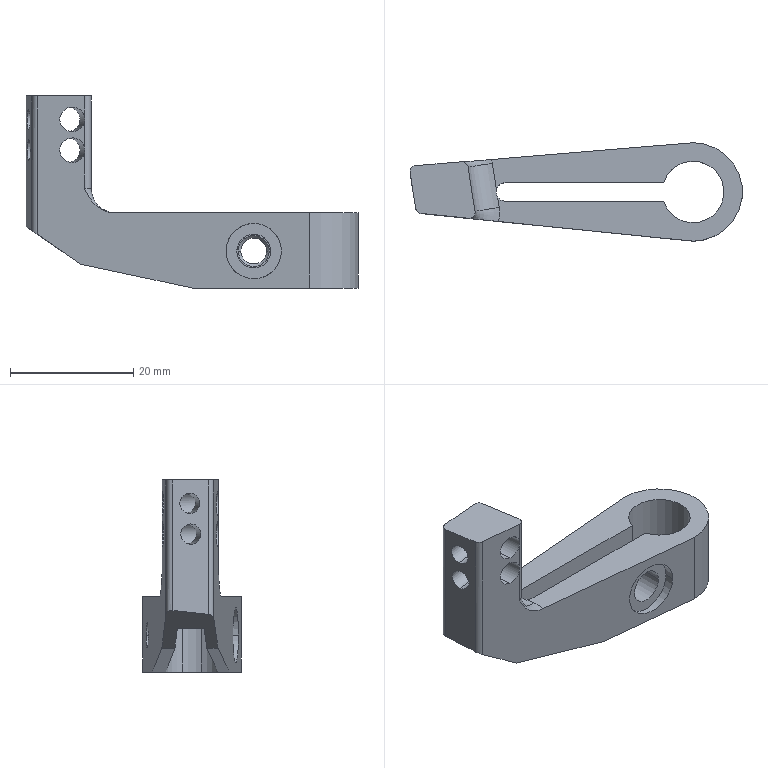CAM job | Mastercam | mm | 2 operations | part box 60.8 x 23.13 x 31.2
1. 3D High Speed (Dynamic OptiRough) | 9 - 8 平铣刀
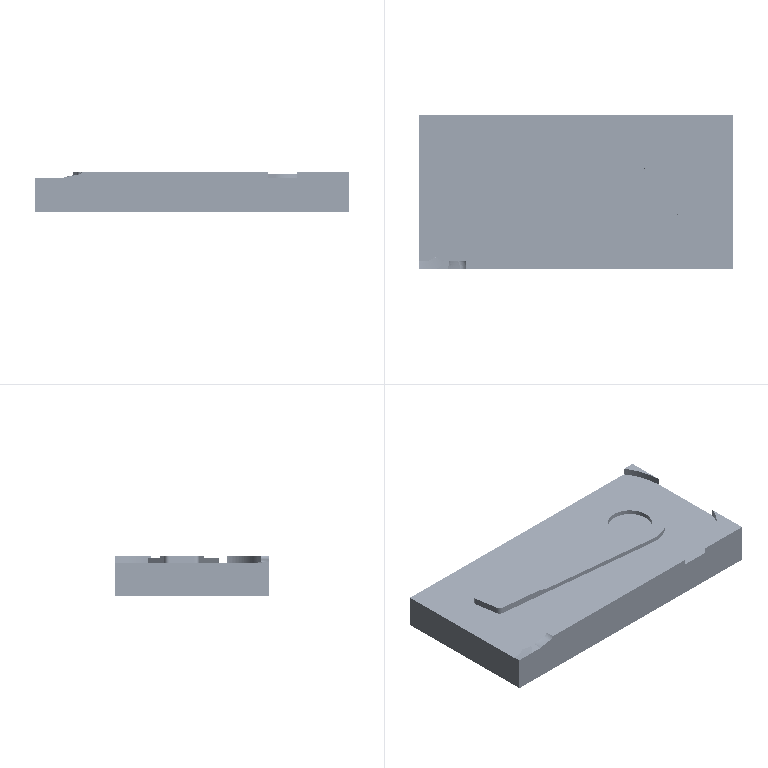2. Contour (Ramp) | 7 - 3 平铣刀